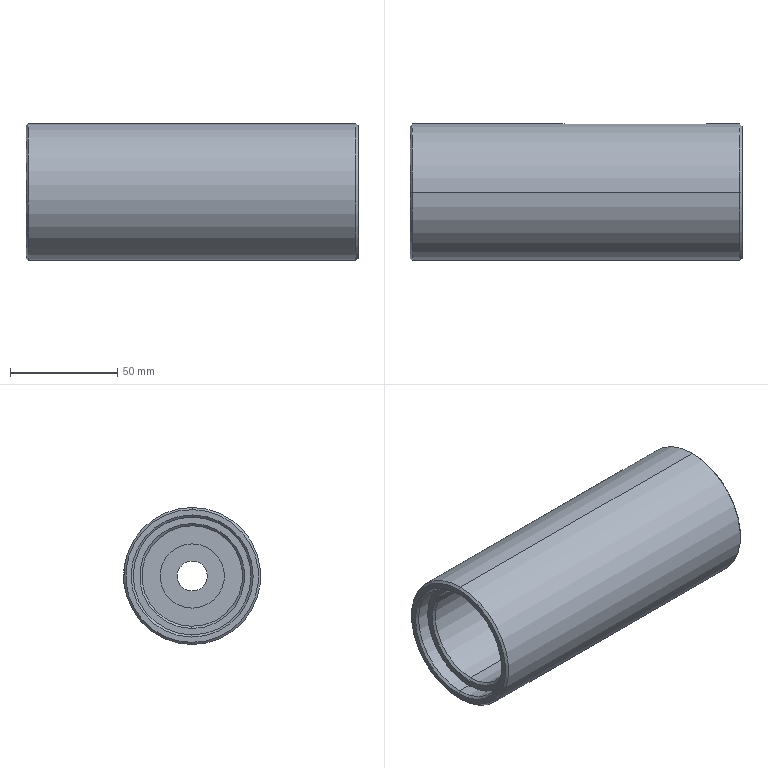Component | SolidWorks | 4-12-12ClampingAxisAssembly-1_4-12-2TelescopicAxis-1 | 1 solid | 28 faces | box 155 x 64 x 64 mm | volume 313641 mm3 | cylinder 12 | cone 8 | plane 8 | commonest cylinder face diameters 14 x2 64 x2 55 x2 47 x2 30 x2 8 x2
build123d program:
from build123d import *

# Parameters (mm, degrees)
HOLE_WIZARD_M16_1_5_D = 14
CHAMFER1_SIZE         = 1
CHAMFER2_SIZE         = 1
CUT_EXTRUDE1_DEPTH    = 4


with BuildPart() as part:
    # Sketch1 → Revolve1 (revolve)
    with BuildSketch(Plane(origin=(0, 0, 0), x_dir=(1, 0, 0), z_dir=(0, 1, 0)), mode=Mode.PRIVATE) as revolve1_sk:
        Polygon((0, 27.5), (0, 32), (155, 32), (155, 0), (104, 0), (104, 15), (94, 15), (94, 23.5), (7, 23.5), (7, 27.5), align=None)
    revolve(revolve1_sk.sketch.rotate(Axis((0, 0, 0), (1, 0, 0)), 180), axis=Axis((0, 0, 0), (1, 0, 0)))

    # Hole Wizard M16 _1.5 (through all)
    with Locations(Plane(origin=(155, 0, 0), x_dir=(0, 0, -1), z_dir=(1, 0, 0))):
        with Locations((0, 0)):
            Hole(HOLE_WIZARD_M16_1_5_D / 2)

    # Chamfer1
    chamfer1_edges = [part.edges().sort_by_distance(p)[0] for p in [
        (0, 0, -32),
        (0, 0, -27.5),
        (7, 0, -23.5),
    ]]
    chamfer(chamfer1_edges, length=CHAMFER1_SIZE)

    # Chamfer2
    chamfer2_edges = [part.edges().sort_by_distance(p)[0] for p in [
        (155, 0, -32),
    ]]
    chamfer(chamfer2_edges, length=CHAMFER2_SIZE)

    # Sketch4 → Cut-Extrude1 (cut)
    with BuildSketch(Plane(origin=(0, 32, 0), x_dir=(-1, 0, 0), z_dir=(0, 1, 0))):
        with BuildLine():
            Line((-136, 4), (-74, 4))
            ThreePointArc((-74, 4), (-70, 0), (-74, -4))
            Line((-74, -4), (-136, -4))
            ThreePointArc((-136, -4), (-140, 0), (-136, 4))
        make_face()
    extrude(amount=-CUT_EXTRUDE1_DEPTH, mode=Mode.SUBTRACT)


solid = part.part

# Placed as in the assembly
solid = solid.moved(Location((-132.809, -4.181, 0), (0.4514, 0, 0)))
STEP:
#1=COLOUR_RGB('',0.7922,0.8196,0.9333);
#2=FILL_AREA_STYLE_COLOUR('',#1);
#3=FILL_AREA_STYLE('',(#2));
#4=SURFACE_STYLE_FILL_AREA(#3);
#5=SURFACE_SIDE_STYLE('',(#4));
#6=SURFACE_STYLE_USAGE(.BOTH.,#5);
#7=PRESENTATION_STYLE_ASSIGNMENT((#6));
#8=CARTESIAN_POINT('',(0.8737,-0.155,-1.22));
#9=VERTEX_POINT('',#8);
#10=CARTESIAN_POINT('',(0.8737,-0.1742,1.22));
#11=VERTEX_POINT('',#10);
#12=CARTESIAN_POINT('',(0.8737,-0.1646,0.));
#13=DIRECTION('',(1.,0.,0.));
#14=DIRECTION('',(0.,-0.007878,1.));
#15=AXIS2_PLACEMENT_3D('',#12,#13,#14);
#16=CIRCLE('',#15,1.22);
#17=EDGE_CURVE('',#9,#11,#16,.T.);
#18=ORIENTED_EDGE('',*,*,#17,.F.);
#19=CARTESIAN_POINT('',(0.8343,-0.1547,-1.26));
#20=VERTEX_POINT('',#19);
#21=CARTESIAN_POINT('',(0.8343,-0.1547,-1.26));
#22=DIRECTION('',(-0.7071,0.005571,-0.7071));
#23=VECTOR('',#22,39.37);
#24=LINE('',#21,#23);
#25=EDGE_CURVE('',#9,#20,#24,.T.);
#26=ORIENTED_EDGE('',*,*,#25,.T.);
#27=CARTESIAN_POINT('',(0.8343,-0.1745,1.26));
#28=VERTEX_POINT('',#27);
#29=CARTESIAN_POINT('',(0.8343,-0.1646,0.));
#30=DIRECTION('',(-1.,-0.,-0.));
#31=DIRECTION('',(0.,-0.007878,1.));
#32=AXIS2_PLACEMENT_3D('',#29,#30,#31);
#33=CIRCLE('',#32,1.26);
#34=EDGE_CURVE('',#28,#20,#33,.T.);
#35=ORIENTED_EDGE('',*,*,#34,.F.);
#36=CARTESIAN_POINT('',(0.8343,-0.1745,1.26));
#37=DIRECTION('',(-0.7071,-0.005571,0.7071));
#38=VECTOR('',#37,39.37);
#39=LINE('',#36,#38);
#40=EDGE_CURVE('',#11,#28,#39,.T.);
#41=ORIENTED_EDGE('',*,*,#40,.F.);
#42=EDGE_LOOP('',(#18,#26,#35,#41));
#43=FACE_OUTER_BOUND('',#42,.T.);
#44=CARTESIAN_POINT('',(0.8343,-0.1646,0.));
#45=DIRECTION('',(-1.,-0.,-0.));
#46=DIRECTION('',(0.,-0.007878,1.));
#47=AXIS2_PLACEMENT_3D('',#44,#45,#46);
#48=CONICAL_SURFACE('',#47,1.26,0.7854);
#49=ADVANCED_FACE('',(#43),#48,.T.);
#50=CARTESIAN_POINT('',(-5.229,-0.1742,1.22));
#51=VERTEX_POINT('',#50);
#52=CARTESIAN_POINT('',(-5.229,-0.155,-1.22));
#53=VERTEX_POINT('',#52);
#54=CARTESIAN_POINT('',(-5.229,-0.1646,0.));
#55=DIRECTION('',(-1.,-0.,-0.));
#56=DIRECTION('',(0.,0.007878,-1.));
#57=AXIS2_PLACEMENT_3D('',#54,#55,#56);
#58=CIRCLE('',#57,1.22);
#59=EDGE_CURVE('',#51,#53,#58,.T.);
#60=ORIENTED_EDGE('',*,*,#59,.F.);
#61=CARTESIAN_POINT('',(-5.189,-0.1745,1.26));
#62=VERTEX_POINT('',#61);
#63=CARTESIAN_POINT('',(-5.229,-0.1742,1.22));
#64=DIRECTION('',(0.7071,-0.005571,0.7071));
#65=VECTOR('',#64,39.37);
#66=LINE('',#63,#65);
#67=EDGE_CURVE('',#51,#62,#66,.T.);
#68=ORIENTED_EDGE('',*,*,#67,.T.);
#69=CARTESIAN_POINT('',(-5.189,-0.1547,-1.26));
#70=VERTEX_POINT('',#69);
#71=CARTESIAN_POINT('',(-5.189,-0.1646,0.));
#72=DIRECTION('',(1.,0.,0.));
#73=DIRECTION('',(0.,0.007878,-1.));
#74=AXIS2_PLACEMENT_3D('',#71,#72,#73);
#75=CIRCLE('',#74,1.26);
#76=EDGE_CURVE('',#70,#62,#75,.T.);
#77=ORIENTED_EDGE('',*,*,#76,.F.);
#78=CARTESIAN_POINT('',(-5.229,-0.155,-1.22));
#79=DIRECTION('',(0.7071,0.005571,-0.7071));
#80=VECTOR('',#79,39.37);
#81=LINE('',#78,#80);
#82=EDGE_CURVE('',#53,#70,#81,.T.);
#83=ORIENTED_EDGE('',*,*,#82,.F.);
#84=EDGE_LOOP('',(#60,#68,#77,#83));
#85=FACE_OUTER_BOUND('',#84,.T.);
#86=CARTESIAN_POINT('',(-5.229,-0.1646,0.));
#87=DIRECTION('',(1.,0.,0.));
#88=DIRECTION('',(0.,0.007878,-1.));
#89=AXIS2_PLACEMENT_3D('',#86,#87,#88);
#90=CONICAL_SURFACE('',#89,1.22,0.7854);
#91=ADVANCED_FACE('',(#85),#90,.T.);
#92=CARTESIAN_POINT('',(-5.189,-0.1561,-1.083));
#93=VERTEX_POINT('',#92);
#94=CARTESIAN_POINT('',(-5.189,-0.1731,1.083));
#95=VERTEX_POINT('',#94);
#96=CARTESIAN_POINT('',(-5.189,-0.1646,0.));
#97=DIRECTION('',(-1.,-0.,-0.));
#98=DIRECTION('',(0.,0.007878,-1.));
#99=AXIS2_PLACEMENT_3D('',#96,#97,#98);
#100=CIRCLE('',#99,1.083);
#101=EDGE_CURVE('',#93,#95,#100,.T.);
#102=ORIENTED_EDGE('',*,*,#101,.F.);
#103=CARTESIAN_POINT('',(-5.229,-0.1558,-1.122));
#104=VERTEX_POINT('',#103);
#105=CARTESIAN_POINT('',(-5.189,-0.1561,-1.083));
#106=DIRECTION('',(-0.7071,0.005571,-0.7071));
#107=VECTOR('',#106,39.37);
#108=LINE('',#105,#107);
#109=EDGE_CURVE('',#93,#104,#108,.T.);
#110=ORIENTED_EDGE('',*,*,#109,.T.);
#111=CARTESIAN_POINT('',(-5.229,-0.1734,1.122));
#112=VERTEX_POINT('',#111);
#113=CARTESIAN_POINT('',(-5.229,-0.1646,0.));
#114=DIRECTION('',(1.,0.,0.));
#115=DIRECTION('',(0.,0.007878,-1.));
#116=AXIS2_PLACEMENT_3D('',#113,#114,#115);
#117=CIRCLE('',#116,1.122);
#118=EDGE_CURVE('',#112,#104,#117,.T.);
#119=ORIENTED_EDGE('',*,*,#118,.F.);
#120=CARTESIAN_POINT('',(-5.189,-0.1731,1.083));
#121=DIRECTION('',(-0.7071,-0.005571,0.7071));
#122=VECTOR('',#121,39.37);
#123=LINE('',#120,#122);
#124=EDGE_CURVE('',#95,#112,#123,.T.);
#125=ORIENTED_EDGE('',*,*,#124,.F.);
#126=EDGE_LOOP('',(#102,#110,#119,#125));
#127=FACE_OUTER_BOUND('',#126,.T.);
#128=CARTESIAN_POINT('',(-5.189,-0.1646,0.));
#129=DIRECTION('',(-1.,-0.,-0.));
#130=DIRECTION('',(0.,-0.007878,1.));
#131=AXIS2_PLACEMENT_3D('',#128,#129,#130);
#132=CONICAL_SURFACE('',#131,1.083,0.7854);
#133=ADVANCED_FACE('',(#127),#132,.F.);
#134=CARTESIAN_POINT('',(-4.914,-0.1573,-0.9252));
#135=VERTEX_POINT('',#134);
#136=CARTESIAN_POINT('',(-4.914,-0.1719,0.9252));
#137=VERTEX_POINT('',#136);
#138=CARTESIAN_POINT('',(-4.914,-0.1646,0.));
#139=DIRECTION('',(-1.,-0.,-0.));
#140=DIRECTION('',(0.,0.007878,-1.));
#141=AXIS2_PLACEMENT_3D('',#138,#139,#140);
#142=CIRCLE('',#141,0.9252);
#143=EDGE_CURVE('',#135,#137,#142,.T.);
#144=ORIENTED_EDGE('',*,*,#143,.F.);
#145=CARTESIAN_POINT('',(-4.953,-0.157,-0.9645));
#146=VERTEX_POINT('',#145);
#147=CARTESIAN_POINT('',(-4.914,-0.1573,-0.9252));
#148=DIRECTION('',(-0.7071,0.005571,-0.7071));
#149=VECTOR('',#148,39.37);
#150=LINE('',#147,#149);
#151=EDGE_CURVE('',#135,#146,#150,.T.);
#152=ORIENTED_EDGE('',*,*,#151,.T.);
#153=CARTESIAN_POINT('',(-4.953,-0.1722,0.9645));
#154=VERTEX_POINT('',#153);
#155=CARTESIAN_POINT('',(-4.953,-0.1646,0.));
#156=DIRECTION('',(1.,0.,0.));
#157=DIRECTION('',(0.,0.007878,-1.));
#158=AXIS2_PLACEMENT_3D('',#155,#156,#157);
#159=CIRCLE('',#158,0.9646);
#160=EDGE_CURVE('',#154,#146,#159,.T.);
#161=ORIENTED_EDGE('',*,*,#160,.F.);
#162=CARTESIAN_POINT('',(-4.914,-0.1719,0.9252));
#163=DIRECTION('',(-0.7071,-0.005571,0.7071));
#164=VECTOR('',#163,39.37);
#165=LINE('',#162,#164);
#166=EDGE_CURVE('',#137,#154,#165,.T.);
#167=ORIENTED_EDGE('',*,*,#166,.F.);
#168=EDGE_LOOP('',(#144,#152,#161,#167));
#169=FACE_OUTER_BOUND('',#168,.T.);
#170=CARTESIAN_POINT('',(-4.914,-0.1646,0.));
#171=DIRECTION('',(-1.,-0.,-0.));
#172=DIRECTION('',(0.,-0.007878,1.));
#173=AXIS2_PLACEMENT_3D('',#170,#171,#172);
#174=CONICAL_SURFACE('',#173,0.9252,0.7854);
#175=ADVANCED_FACE('',(#169),#174,.F.);
#176=CARTESIAN_POINT('',(-1.134,-0.1668,0.2756));
#177=VERTEX_POINT('',#176);
#178=CARTESIAN_POINT('',(-1.134,-0.1624,-0.2756));
#179=VERTEX_POINT('',#178);
#180=CARTESIAN_POINT('',(-1.134,-0.1646,0.));
#181=DIRECTION('',(1.,0.,0.));
#182=DIRECTION('',(0.,0.007878,-1.));
#183=AXIS2_PLACEMENT_3D('',#180,#181,#182);
#184=CIRCLE('',#183,0.2756);
#185=EDGE_CURVE('',#177,#179,#184,.T.);
#186=ORIENTED_EDGE('',*,*,#185,.F.);
#187=CARTESIAN_POINT('',(0.8737,-0.1668,0.2756));
#188=VERTEX_POINT('',#187);
#189=CARTESIAN_POINT('',(0.8737,-0.1668,0.2756));
#190=DIRECTION('',(1.,0.,0.));
#191=VECTOR('',#190,39.37);
#192=LINE('',#189,#191);
#193=EDGE_CURVE('',#177,#188,#192,.T.);
#194=ORIENTED_EDGE('',*,*,#193,.T.);
#195=CARTESIAN_POINT('',(0.8737,-0.1624,-0.2756));
#196=VERTEX_POINT('',#195);
#197=CARTESIAN_POINT('',(0.8737,-0.1646,0.));
#198=DIRECTION('',(1.,0.,0.));
#199=DIRECTION('',(0.,0.007878,-1.));
#200=AXIS2_PLACEMENT_3D('',#197,#198,#199);
#201=CIRCLE('',#200,0.2756);
#202=EDGE_CURVE('',#188,#196,#201,.T.);
#203=ORIENTED_EDGE('',*,*,#202,.T.);
#204=CARTESIAN_POINT('',(0.8737,-0.1624,-0.2756));
#205=DIRECTION('',(1.,0.,0.));
#206=VECTOR('',#205,39.37);
#207=LINE('',#204,#206);
#208=EDGE_CURVE('',#179,#196,#207,.T.);
#209=ORIENTED_EDGE('',*,*,#208,.F.);
#210=EDGE_LOOP('',(#186,#194,#203,#209));
#211=FACE_OUTER_BOUND('',#210,.T.);
#212=CARTESIAN_POINT('',(0.8737,-0.1646,0.));
#213=DIRECTION('',(1.,0.,0.));
#214=DIRECTION('',(0.,0.007878,-1.));
#215=AXIS2_PLACEMENT_3D('',#212,#213,#214);
#216=CYLINDRICAL_SURFACE('',#215,0.2756);
#217=ADVANCED_FACE('',(#211),#216,.F.);
#218=CARTESIAN_POINT('',(0.1256,1.084,0.1673));
#219=VERTEX_POINT('',#218);
#220=CARTESIAN_POINT('',(-2.315,1.084,0.1673));
#221=VERTEX_POINT('',#220);
#222=CARTESIAN_POINT('',(-5.229,1.084,0.1673));
#223=DIRECTION('',(-1.,-0.,-0.));
#224=VECTOR('',#223,39.37);
#225=LINE('',#222,#224);
#226=EDGE_CURVE('',#219,#221,#225,.T.);
#227=ORIENTED_EDGE('',*,*,#226,.T.);
#228=CARTESIAN_POINT('',(-2.315,1.087,-0.1476));
#229=VERTEX_POINT('',#228);
#230=CARTESIAN_POINT('',(-2.315,1.084,0.1673));
#231=CARTESIAN_POINT('',(-2.326,1.084,0.1673));
#232=CARTESIAN_POINT('',(-2.336,1.084,0.1663));
#233=CARTESIAN_POINT('',(-2.356,1.085,0.1623));
#234=CARTESIAN_POINT('',(-2.366,1.085,0.1593));
#235=CARTESIAN_POINT('',(-2.385,1.086,0.1514));
#236=CARTESIAN_POINT('',(-2.394,1.087,0.1465));
#237=CARTESIAN_POINT('',(-2.411,1.088,0.1351));
#238=CARTESIAN_POINT('',(-2.419,1.089,0.1285));
#239=CARTESIAN_POINT('',(-2.434,1.09,0.114));
#240=CARTESIAN_POINT('',(-2.44,1.091,0.1061));
#241=CARTESIAN_POINT('',(-2.452,1.092,0.08887));
#242=CARTESIAN_POINT('',(-2.457,1.093,0.07973));
#243=CARTESIAN_POINT('',(-2.465,1.094,0.0608));
#244=CARTESIAN_POINT('',(-2.468,1.094,0.05087));
#245=CARTESIAN_POINT('',(-2.472,1.095,0.03054));
#246=CARTESIAN_POINT('',(-2.473,1.095,0.02032));
#247=CARTESIAN_POINT('',(-2.473,1.095,-0.0002398));
#248=CARTESIAN_POINT('',(-2.472,1.095,-0.01068));
#249=CARTESIAN_POINT('',(-2.468,1.095,-0.03089));
#250=CARTESIAN_POINT('',(-2.465,1.095,-0.04071));
#251=CARTESIAN_POINT('',(-2.457,1.094,-0.0598));
#252=CARTESIAN_POINT('',(-2.452,1.093,-0.06901));
#253=CARTESIAN_POINT('',(-2.441,1.092,-0.08607));
#254=CARTESIAN_POINT('',(-2.434,1.092,-0.09404));
#255=CARTESIAN_POINT('',(-2.419,1.091,-0.1087));
#256=CARTESIAN_POINT('',(-2.411,1.09,-0.1153));
#257=CARTESIAN_POINT('',(-2.394,1.089,-0.1267));
#258=CARTESIAN_POINT('',(-2.385,1.088,-0.1316));
#259=CARTESIAN_POINT('',(-2.366,1.087,-0.1395));
#260=CARTESIAN_POINT('',(-2.356,1.087,-0.1425));
#261=CARTESIAN_POINT('',(-2.336,1.087,-0.1466));
#262=CARTESIAN_POINT('',(-2.326,1.087,-0.1476));
#263=CARTESIAN_POINT('',(-2.315,1.087,-0.1476));
#264=B_SPLINE_CURVE_WITH_KNOTS('',3,(#230,#231,#232,#233,#234,#235,#236,#237,#238,#239,#240,#241,#242,#243,#244,#245,#246,#247,#248,#249,#250,#251,#252,#253,#254,#255,#256,#257,#258,#259,#260,#261,#262,#263),.UNSPECIFIED.,.F.,.F.,(4,2,2,2,2,2,2,2,2,2,2,2,2,2,2,2,4),(0.,0.0007822,0.001564,0.002347,0.003129,0.003911,0.004693,0.005475,0.006258,0.00704,0.007822,0.008604,0.009386,0.01017,0.01095,0.01173,0.01252),.UNSPECIFIED.);
#265=EDGE_CURVE('',#221,#229,#264,.T.);
#266=ORIENTED_EDGE('',*,*,#265,.T.);
#267=CARTESIAN_POINT('',(0.1256,1.087,-0.1476));
#268=VERTEX_POINT('',#267);
#269=CARTESIAN_POINT('',(-5.229,1.087,-0.1476));
#270=DIRECTION('',(1.,0.,0.));
#271=VECTOR('',#270,39.37);
#272=LINE('',#269,#271);
#273=EDGE_CURVE('',#229,#268,#272,.T.);
#274=ORIENTED_EDGE('',*,*,#273,.T.);
#275=CARTESIAN_POINT('',(0.1256,1.087,-0.1476));
#276=CARTESIAN_POINT('',(0.136,1.087,-0.1476));
#277=CARTESIAN_POINT('',(0.1463,1.087,-0.1466));
#278=CARTESIAN_POINT('',(0.1664,1.087,-0.1426));
#279=CARTESIAN_POINT('',(0.1764,1.087,-0.1396));
#280=CARTESIAN_POINT('',(0.1955,1.088,-0.1316));
#281=CARTESIAN_POINT('',(0.2045,1.089,-0.1268));
#282=CARTESIAN_POINT('',(0.2216,1.09,-0.1154));
#283=CARTESIAN_POINT('',(0.2297,1.091,-0.1087));
#284=CARTESIAN_POINT('',(0.2442,1.092,-0.0942));
#285=CARTESIAN_POINT('',(0.2508,1.092,-0.08628));
#286=CARTESIAN_POINT('',(0.2623,1.093,-0.06906));
#287=CARTESIAN_POINT('',(0.2672,1.094,-0.05991));
#288=CARTESIAN_POINT('',(0.275,1.095,-0.04096));
#289=CARTESIAN_POINT('',(0.278,1.095,-0.03103));
#290=CARTESIAN_POINT('',(0.2821,1.095,-0.01069));
#291=CARTESIAN_POINT('',(0.2831,1.095,-0.0004692));
#292=CARTESIAN_POINT('',(0.2831,1.095,0.02009));
#293=CARTESIAN_POINT('',(0.2821,1.095,0.03053));
#294=CARTESIAN_POINT('',(0.2781,1.094,0.05073));
#295=CARTESIAN_POINT('',(0.2751,1.094,0.06055));
#296=CARTESIAN_POINT('',(0.2672,1.093,0.07962));
#297=CARTESIAN_POINT('',(0.2623,1.092,0.08882));
#298=CARTESIAN_POINT('',(0.2509,1.091,0.1059));
#299=CARTESIAN_POINT('',(0.2444,1.09,0.1138));
#300=CARTESIAN_POINT('',(0.2297,1.089,0.1285));
#301=CARTESIAN_POINT('',(0.2218,1.088,0.135));
#302=CARTESIAN_POINT('',(0.2047,1.087,0.1464));
#303=CARTESIAN_POINT('',(0.1955,1.086,0.1514));
#304=CARTESIAN_POINT('',(0.1765,1.085,0.1593));
#305=CARTESIAN_POINT('',(0.1667,1.085,0.1622));
#306=CARTESIAN_POINT('',(0.1465,1.084,0.1663));
#307=CARTESIAN_POINT('',(0.136,1.084,0.1673));
#308=CARTESIAN_POINT('',(0.1256,1.084,0.1673));
#309=B_SPLINE_CURVE_WITH_KNOTS('',3,(#275,#276,#277,#278,#279,#280,#281,#282,#283,#284,#285,#286,#287,#288,#289,#290,#291,#292,#293,#294,#295,#296,#297,#298,#299,#300,#301,#302,#303,#304,#305,#306,#307,#308),.UNSPECIFIED.,.F.,.F.,(4,2,2,2,2,2,2,2,2,2,2,2,2,2,2,2,4),(0.,0.0007822,0.001564,0.002347,0.003129,0.003911,0.004693,0.005475,0.006258,0.00704,0.007822,0.008604,0.009386,0.01017,0.01095,0.01173,0.01252),.UNSPECIFIED.);
#310=EDGE_CURVE('',#268,#219,#309,.T.);
#311=ORIENTED_EDGE('',*,*,#310,.T.);
#312=EDGE_LOOP('',(#227,#266,#274,#311));
#313=FACE_BOUND('',#312,.T.);
#314=ORIENTED_EDGE('',*,*,#34,.T.);
#315=CARTESIAN_POINT('',(-5.229,-0.1547,-1.26));
#316=DIRECTION('',(-1.,-0.,-0.));
#317=VECTOR('',#316,39.37);
#318=LINE('',#315,#317);
#319=EDGE_CURVE('',#20,#70,#318,.T.);
#320=ORIENTED_EDGE('',*,*,#319,.T.);
#321=ORIENTED_EDGE('',*,*,#76,.T.);
#322=CARTESIAN_POINT('',(-5.229,-0.1745,1.26));
#323=DIRECTION('',(-1.,-0.,-0.));
#324=VECTOR('',#323,39.37);
#325=LINE('',#322,#324);
#326=EDGE_CURVE('',#28,#62,#325,.T.);
#327=ORIENTED_EDGE('',*,*,#326,.F.);
#328=EDGE_LOOP('',(#314,#320,#321,#327));
#329=FACE_OUTER_BOUND('',#328,.T.);
#330=CARTESIAN_POINT('',(-5.229,-0.1646,0.));
#331=DIRECTION('',(-1.,-0.,-0.));
#332=DIRECTION('',(0.,-0.007878,1.));
#333=AXIS2_PLACEMENT_3D('',#330,#331,#332);
#334=CYLINDRICAL_SURFACE('',#333,1.26);
#335=ADVANCED_FACE('',(#313,#329),#334,.T.);
#336=CARTESIAN_POINT('',(-4.953,-0.1561,-1.083));
#337=VERTEX_POINT('',#336);
#338=CARTESIAN_POINT('',(-4.953,-0.1731,1.083));
#339=VERTEX_POINT('',#338);
#340=CARTESIAN_POINT('',(-4.953,-0.1646,0.));
#341=DIRECTION('',(-1.,-0.,-0.));
#342=DIRECTION('',(0.,-0.007878,1.));
#343=AXIS2_PLACEMENT_3D('',#340,#341,#342);
#344=CIRCLE('',#343,1.083);
#345=EDGE_CURVE('',#337,#339,#344,.T.);
#346=ORIENTED_EDGE('',*,*,#345,.F.);
#347=CARTESIAN_POINT('',(-5.229,-0.1561,-1.083));
#348=DIRECTION('',(-1.,-0.,-0.));
#349=VECTOR('',#348,39.37);
#350=LINE('',#347,#349);
#351=EDGE_CURVE('',#337,#93,#350,.T.);
#352=ORIENTED_EDGE('',*,*,#351,.T.);
#353=ORIENTED_EDGE('',*,*,#101,.T.);
#354=CARTESIAN_POINT('',(-5.229,-0.1731,1.083));
#355=DIRECTION('',(-1.,-0.,-0.));
#356=VECTOR('',#355,39.37);
#357=LINE('',#354,#356);
#358=EDGE_CURVE('',#339,#95,#357,.T.);
#359=ORIENTED_EDGE('',*,*,#358,.F.);
#360=EDGE_LOOP('',(#346,#352,#353,#359));
#361=FACE_OUTER_BOUND('',#360,.T.);
#362=CARTESIAN_POINT('',(-5.229,-0.1646,0.));
#363=DIRECTION('',(-1.,-0.,-0.));
#364=DIRECTION('',(0.,-0.007878,1.));
#365=AXIS2_PLACEMENT_3D('',#362,#363,#364);
#366=CYLINDRICAL_SURFACE('',#365,1.083);
#367=ADVANCED_FACE('',(#361),#366,.F.);
#368=CARTESIAN_POINT('',(-1.528,-0.1573,-0.9252));
#369=VERTEX_POINT('',#368);
#370=CARTESIAN_POINT('',(-1.528,-0.1719,0.9252));
#371=VERTEX_POINT('',#370);
#372=CARTESIAN_POINT('',(-1.528,-0.1646,0.));
#373=DIRECTION('',(-1.,-0.,-0.));
#374=DIRECTION('',(0.,-0.007878,1.));
#375=AXIS2_PLACEMENT_3D('',#372,#373,#374);
#376=CIRCLE('',#375,0.9252);
#377=EDGE_CURVE('',#369,#371,#376,.T.);
#378=ORIENTED_EDGE('',*,*,#377,.F.);
#379=CARTESIAN_POINT('',(-5.229,-0.1573,-0.9252));
#380=DIRECTION('',(-1.,-0.,-0.));
#381=VECTOR('',#380,39.37);
#382=LINE('',#379,#381);
#383=EDGE_CURVE('',#369,#135,#382,.T.);
#384=ORIENTED_EDGE('',*,*,#383,.T.);
#385=ORIENTED_EDGE('',*,*,#143,.T.);
#386=CARTESIAN_POINT('',(-5.229,-0.1719,0.9252));
#387=DIRECTION('',(-1.,-0.,-0.));
#388=VECTOR('',#387,39.37);
#389=LINE('',#386,#388);
#390=EDGE_CURVE('',#371,#137,#389,.T.);
#391=ORIENTED_EDGE('',*,*,#390,.F.);
#392=EDGE_LOOP('',(#378,#384,#385,#391));
#393=FACE_OUTER_BOUND('',#392,.T.);
#394=CARTESIAN_POINT('',(-5.229,-0.1646,0.));
#395=DIRECTION('',(-1.,-0.,-0.));
#396=DIRECTION('',(0.,-0.007878,1.));
#397=AXIS2_PLACEMENT_3D('',#394,#395,#396);
#398=CYLINDRICAL_SURFACE('',#397,0.9252);
#399=ADVANCED_FACE('',(#393),#398,.F.);
#400=CARTESIAN_POINT('',(-1.134,-0.16,-0.5905));
#401=VERTEX_POINT('',#400);
#402=CARTESIAN_POINT('',(-1.134,-0.1693,0.5905));
#403=VERTEX_POINT('',#402);
#404=CARTESIAN_POINT('',(-1.134,-0.1646,0.));
#405=DIRECTION('',(-1.,-0.,-0.));
#406=DIRECTION('',(0.,-0.007878,1.));
#407=AXIS2_PLACEMENT_3D('',#404,#405,#406);
#408=CIRCLE('',#407,0.5906);
#409=EDGE_CURVE('',#401,#403,#408,.T.);
#410=ORIENTED_EDGE('',*,*,#409,.F.);
#411=CARTESIAN_POINT('',(-1.528,-0.16,-0.5905));
#412=VERTEX_POINT('',#411);
#413=CARTESIAN_POINT('',(-5.229,-0.16,-0.5905));
#414=DIRECTION('',(-1.,-0.,-0.));
#415=VECTOR('',#414,39.37);
#416=LINE('',#413,#415);
#417=EDGE_CURVE('',#401,#412,#416,.T.);
#418=ORIENTED_EDGE('',*,*,#417,.T.);
#419=CARTESIAN_POINT('',(-1.528,-0.1693,0.5905));
#420=VERTEX_POINT('',#419);
#421=CARTESIAN_POINT('',(-1.528,-0.1646,0.));
#422=DIRECTION('',(-1.,-0.,-0.));
#423=DIRECTION('',(0.,-0.007878,1.));
#424=AXIS2_PLACEMENT_3D('',#421,#422,#423);
#425=CIRCLE('',#424,0.5906);
#426=EDGE_CURVE('',#412,#420,#425,.T.);
#427=ORIENTED_EDGE('',*,*,#426,.T.);
#428=CARTESIAN_POINT('',(-5.229,-0.1693,0.5905));
#429=DIRECTION('',(-1.,-0.,-0.));
#430=VECTOR('',#429,39.37);
#431=LINE('',#428,#430);
#432=EDGE_CURVE('',#403,#420,#431,.T.);
#433=ORIENTED_EDGE('',*,*,#432,.F.);
#434=EDGE_LOOP('',(#410,#418,#427,#433));
#435=FACE_OUTER_BOUND('',#434,.T.);
#436=CARTESIAN_POINT('',(-5.229,-0.1646,0.));
#437=DIRECTION('',(-1.,-0.,-0.));
#438=DIRECTION('',(0.,-0.007878,1.));
#439=AXIS2_PLACEMENT_3D('',#436,#437,#438);
#440=CYLINDRICAL_SURFACE('',#439,0.5906);
#441=ADVANCED_FACE('',(#435),#440,.F.);
#442=CARTESIAN_POINT('',(-1.134,-0.1646,0.));
#443=DIRECTION('',(1.,0.,0.));
#444=DIRECTION('',(0.,0.007878,-1.));
#445=AXIS2_PLACEMENT_3D('',#442,#443,#444);
#446=CIRCLE('',#445,0.2756);
#447=EDGE_CURVE('',#179,#177,#446,.T.);
#448=ORIENTED_EDGE('',*,*,#447,.T.);
#449=ORIENTED_EDGE('',*,*,#185,.T.);
#450=EDGE_LOOP('',(#448,#449));
#451=FACE_BOUND('',#450,.T.);
#452=CARTESIAN_POINT('',(-1.134,-0.1646,0.));
#453=DIRECTION('',(-1.,-0.,-0.));
#454=DIRECTION('',(0.,-0.007878,1.));
#455=AXIS2_PLACEMENT_3D('',#452,#453,#454);
#456=CIRCLE('',#455,0.5906);
#457=EDGE_CURVE('',#403,#401,#456,.T.);
#458=ORIENTED_EDGE('',*,*,#457,.T.);
#459=ORIENTED_EDGE('',*,*,#409,.T.);
#460=EDGE_LOOP('',(#458,#459));
#461=FACE_OUTER_BOUND('',#460,.T.);
#462=CARTESIAN_POINT('',(-1.134,-0.1646,0.));
#463=DIRECTION('',(1.,0.,0.));
#464=DIRECTION('',(0.,0.007878,-1.));
#465=AXIS2_PLACEMENT_3D('',#462,#463,#464);
#466=PLANE('',#465);
#467=ADVANCED_FACE('',(#451,#461),#466,.F.);
#468=ORIENTED_EDGE('',*,*,#417,.F.);
#469=ORIENTED_EDGE('',*,*,#457,.F.);
#470=ORIENTED_EDGE('',*,*,#432,.T.);
#471=CARTESIAN_POINT('',(-1.528,-0.1646,0.));
#472=DIRECTION('',(-1.,-0.,-0.));
#473=DIRECTION('',(0.,-0.007878,1.));
#474=AXIS2_PLACEMENT_3D('',#471,#472,#473);
#475=CIRCLE('',#474,0.5906);
#476=EDGE_CURVE('',#420,#412,#475,.T.);
#477=ORIENTED_EDGE('',*,*,#476,.T.);
#478=EDGE_LOOP('',(#468,#469,#470,#477));
#479=FACE_OUTER_BOUND('',#478,.T.);
#480=CARTESIAN_POINT('',(-5.229,-0.1646,0.));
#481=DIRECTION('',(-1.,-0.,-0.));
#482=DIRECTION('',(0.,-0.007878,1.));
#483=AXIS2_PLACEMENT_3D('',#480,#481,#482);
#484=CYLINDRICAL_SURFACE('',#483,0.5906);
#485=ADVANCED_FACE('',(#479),#484,.F.);
#486=ORIENTED_EDGE('',*,*,#476,.F.);
#487=ORIENTED_EDGE('',*,*,#426,.F.);
#488=EDGE_LOOP('',(#486,#487));
#489=FACE_BOUND('',#488,.T.);
#490=CARTESIAN_POINT('',(-1.528,-0.1646,0.));
#491=DIRECTION('',(-1.,-0.,-0.));
#492=DIRECTION('',(0.,-0.007878,1.));
#493=AXIS2_PLACEMENT_3D('',#490,#491,#492);
#494=CIRCLE('',#493,0.9252);
#495=EDGE_CURVE('',#371,#369,#494,.T.);
#496=ORIENTED_EDGE('',*,*,#495,.T.);
#497=ORIENTED_EDGE('',*,*,#377,.T.);
#498=EDGE_LOOP('',(#496,#497));
#499=FACE_OUTER_BOUND('',#498,.T.);
#500=CARTESIAN_POINT('',(-1.528,-0.16,-0.5905));
#501=DIRECTION('',(1.,0.,0.));
#502=DIRECTION('',(0.,0.007878,-1.));
#503=AXIS2_PLACEMENT_3D('',#500,#501,#502);
#504=PLANE('',#503);
#505=ADVANCED_FACE('',(#489,#499),#504,.F.);
#506=ORIENTED_EDGE('',*,*,#383,.F.);
#507=ORIENTED_EDGE('',*,*,#495,.F.);
#508=ORIENTED_EDGE('',*,*,#390,.T.);
#509=CARTESIAN_POINT('',(-4.914,-0.1646,0.));
#510=DIRECTION('',(-1.,-0.,-0.));
#511=DIRECTION('',(0.,0.007878,-1.));
#512=AXIS2_PLACEMENT_3D('',#509,#510,#511);
#513=CIRCLE('',#512,0.9252);
#514=EDGE_CURVE('',#137,#135,#513,.T.);
#515=ORIENTED_EDGE('',*,*,#514,.T.);
#516=EDGE_LOOP('',(#506,#507,#508,#515));
#517=FACE_OUTER_BOUND('',#516,.T.);
#518=CARTESIAN_POINT('',(-5.229,-0.1646,0.));
#519=DIRECTION('',(-1.,-0.,-0.));
#520=DIRECTION('',(0.,-0.007878,1.));
#521=AXIS2_PLACEMENT_3D('',#518,#519,#520);
#522=CYLINDRICAL_SURFACE('',#521,0.9252);
#523=ADVANCED_FACE('',(#517),#522,.F.);
#524=ORIENTED_EDGE('',*,*,#160,.T.);
#525=CARTESIAN_POINT('',(-4.953,-0.1646,0.));
#526=DIRECTION('',(1.,0.,0.));
#527=DIRECTION('',(0.,0.007878,-1.));
#528=AXIS2_PLACEMENT_3D('',#525,#526,#527);
#529=CIRCLE('',#528,0.9646);
#530=EDGE_CURVE('',#146,#154,#529,.T.);
#531=ORIENTED_EDGE('',*,*,#530,.T.);
#532=EDGE_LOOP('',(#524,#531));
#533=FACE_BOUND('',#532,.T.);
#534=CARTESIAN_POINT('',(-4.953,-0.1646,0.));
#535=DIRECTION('',(-1.,-0.,-0.));
#536=DIRECTION('',(0.,-0.007878,1.));
#537=AXIS2_PLACEMENT_3D('',#534,#535,#536);
#538=CIRCLE('',#537,1.083);
#539=EDGE_CURVE('',#339,#337,#538,.T.);
#540=ORIENTED_EDGE('',*,*,#539,.T.);
#541=ORIENTED_EDGE('',*,*,#345,.T.);
#542=EDGE_LOOP('',(#540,#541));
#543=FACE_OUTER_BOUND('',#542,.T.);
#544=CARTESIAN_POINT('',(-4.953,-0.1573,-0.9252));
#545=DIRECTION('',(1.,0.,0.));
#546=DIRECTION('',(0.,0.007878,-1.));
#547=AXIS2_PLACEMENT_3D('',#544,#545,#546);
#548=PLANE('',#547);
#549=ADVANCED_FACE('',(#533,#543),#548,.F.);
#550=ORIENTED_EDGE('',*,*,#351,.F.);
#551=ORIENTED_EDGE('',*,*,#539,.F.);
#552=ORIENTED_EDGE('',*,*,#358,.T.);
#553=CARTESIAN_POINT('',(-5.189,-0.1646,0.));
#554=DIRECTION('',(-1.,-0.,-0.));
#555=DIRECTION('',(0.,0.007878,-1.));
#556=AXIS2_PLACEMENT_3D('',#553,#554,#555);
#557=CIRCLE('',#556,1.083);
#558=EDGE_CURVE('',#95,#93,#557,.T.);
#559=ORIENTED_EDGE('',*,*,#558,.T.);
#560=EDGE_LOOP('',(#550,#551,#552,#559));
#561=FACE_OUTER_BOUND('',#560,.T.);
#562=CARTESIAN_POINT('',(-5.229,-0.1646,0.));
#563=DIRECTION('',(-1.,-0.,-0.));
#564=DIRECTION('',(0.,-0.007878,1.));
#565=AXIS2_PLACEMENT_3D('',#562,#563,#564);
#566=CYLINDRICAL_SURFACE('',#565,1.083);
#567=ADVANCED_FACE('',(#561),#566,.F.);
#568=ORIENTED_EDGE('',*,*,#118,.T.);
#569=CARTESIAN_POINT('',(-5.229,-0.1646,0.));
#570=DIRECTION('',(1.,0.,0.));
#571=DIRECTION('',(0.,0.007878,-1.));
#572=AXIS2_PLACEMENT_3D('',#569,#570,#571);
#573=CIRCLE('',#572,1.122);
#574=EDGE_CURVE('',#104,#112,#573,.T.);
#575=ORIENTED_EDGE('',*,*,#574,.T.);
#576=EDGE_LOOP('',(#568,#575));
#577=FACE_BOUND('',#576,.T.);
#578=CARTESIAN_POINT('',(-5.229,-0.1646,0.));
#579=DIRECTION('',(-1.,-0.,-0.));
#580=DIRECTION('',(0.,0.007878,-1.));
#581=AXIS2_PLACEMENT_3D('',#578,#579,#580);
#582=CIRCLE('',#581,1.22);
#583=EDGE_CURVE('',#53,#51,#582,.T.);
#584=ORIENTED_EDGE('',*,*,#583,.T.);
#585=ORIENTED_EDGE('',*,*,#59,.T.);
#586=EDGE_LOOP('',(#584,#585));
#587=FACE_OUTER_BOUND('',#586,.T.);
#588=CARTESIAN_POINT('',(-5.229,-0.1561,-1.083));
#589=DIRECTION('',(1.,0.,0.));
#590=DIRECTION('',(0.,0.007878,-1.));
#591=AXIS2_PLACEMENT_3D('',#588,#589,#590);
#592=PLANE('',#591);
#593=ADVANCED_FACE('',(#577,#587),#592,.F.);
#594=ORIENTED_EDGE('',*,*,#319,.F.);
#595=CARTESIAN_POINT('',(0.8343,-0.1646,0.));
#596=DIRECTION('',(-1.,-0.,-0.));
#597=DIRECTION('',(0.,-0.007878,1.));
#598=AXIS2_PLACEMENT_3D('',#595,#596,#597);
#599=CIRCLE('',#598,1.26);
#600=EDGE_CURVE('',#20,#28,#599,.T.);
#601=ORIENTED_EDGE('',*,*,#600,.T.);
#602=ORIENTED_EDGE('',*,*,#326,.T.);
#603=CARTESIAN_POINT('',(-5.189,-0.1646,0.));
#604=DIRECTION('',(1.,0.,0.));
#605=DIRECTION('',(0.,0.007878,-1.));
#606=AXIS2_PLACEMENT_3D('',#603,#604,#605);
#607=CIRCLE('',#606,1.26);
#608=EDGE_CURVE('',#62,#70,#607,.T.);
#609=ORIENTED_EDGE('',*,*,#608,.T.);
#610=EDGE_LOOP('',(#594,#601,#602,#609));
#611=FACE_OUTER_BOUND('',#610,.T.);
#612=CARTESIAN_POINT('',(-5.229,-0.1646,0.));
#613=DIRECTION('',(-1.,-0.,-0.));
#614=DIRECTION('',(0.,-0.007878,1.));
#615=AXIS2_PLACEMENT_3D('',#612,#613,#614);
#616=CYLINDRICAL_SURFACE('',#615,1.26);
#617=ADVANCED_FACE('',(#611),#616,.T.);
#618=CARTESIAN_POINT('',(0.8737,-0.1646,0.));
#619=DIRECTION('',(1.,0.,0.));
#620=DIRECTION('',(0.,-0.007878,1.));
#621=AXIS2_PLACEMENT_3D('',#618,#619,#620);
#622=CIRCLE('',#621,1.22);
#623=EDGE_CURVE('',#11,#9,#622,.T.);
#624=ORIENTED_EDGE('',*,*,#623,.T.);
#625=ORIENTED_EDGE('',*,*,#17,.T.);
#626=EDGE_LOOP('',(#624,#625));
#627=FACE_OUTER_BOUND('',#626,.T.);
#628=CARTESIAN_POINT('',(0.8737,-0.1646,0.));
#629=DIRECTION('',(1.,0.,0.));
#630=DIRECTION('',(0.,0.007878,-1.));
#631=AXIS2_PLACEMENT_3D('',#628,#629,#630);
#632=CIRCLE('',#631,0.2756);
#633=EDGE_CURVE('',#196,#188,#632,.T.);
#634=ORIENTED_EDGE('',*,*,#633,.F.);
#635=ORIENTED_EDGE('',*,*,#202,.F.);
#636=EDGE_LOOP('',(#634,#635));
#637=FACE_BOUND('',#636,.T.);
#638=CARTESIAN_POINT('',(0.8737,-0.1547,-1.26));
#639=DIRECTION('',(-1.,-0.,-0.));
#640=DIRECTION('',(-0.,-0.007878,1.));
#641=AXIS2_PLACEMENT_3D('',#638,#639,#640);
#642=PLANE('',#641);
#643=ADVANCED_FACE('',(#627,#637),#642,.F.);
#644=ORIENTED_EDGE('',*,*,#193,.F.);
#645=ORIENTED_EDGE('',*,*,#447,.F.);
#646=ORIENTED_EDGE('',*,*,#208,.T.);
#647=ORIENTED_EDGE('',*,*,#633,.T.);
#648=EDGE_LOOP('',(#644,#645,#646,#647));
#649=FACE_OUTER_BOUND('',#648,.T.);
#650=CARTESIAN_POINT('',(0.8737,-0.1646,0.));
#651=DIRECTION('',(1.,0.,0.));
#652=DIRECTION('',(0.,0.007878,-1.));
#653=AXIS2_PLACEMENT_3D('',#650,#651,#652);
#654=CYLINDRICAL_SURFACE('',#653,0.2756);
#655=ADVANCED_FACE('',(#649),#654,.F.);
#656=ORIENTED_EDGE('',*,*,#151,.F.);
#657=ORIENTED_EDGE('',*,*,#514,.F.);
#658=ORIENTED_EDGE('',*,*,#166,.T.);
#659=ORIENTED_EDGE('',*,*,#530,.F.);
#660=EDGE_LOOP('',(#656,#657,#658,#659));
#661=FACE_OUTER_BOUND('',#660,.T.);
#662=CARTESIAN_POINT('',(-4.914,-0.1646,0.));
#663=DIRECTION('',(-1.,-0.,-0.));
#664=DIRECTION('',(0.,-0.007878,1.));
#665=AXIS2_PLACEMENT_3D('',#662,#663,#664);
#666=CONICAL_SURFACE('',#665,0.9252,0.7854);
#667=ADVANCED_FACE('',(#661),#666,.F.);
#668=ORIENTED_EDGE('',*,*,#109,.F.);
#669=ORIENTED_EDGE('',*,*,#558,.F.);
#670=ORIENTED_EDGE('',*,*,#124,.T.);
#671=ORIENTED_EDGE('',*,*,#574,.F.);
#672=EDGE_LOOP('',(#668,#669,#670,#671));
#673=FACE_OUTER_BOUND('',#672,.T.);
#674=CARTESIAN_POINT('',(-5.189,-0.1646,0.));
#675=DIRECTION('',(-1.,-0.,-0.));
#676=DIRECTION('',(0.,-0.007878,1.));
#677=AXIS2_PLACEMENT_3D('',#674,#675,#676);
#678=CONICAL_SURFACE('',#677,1.083,0.7854);
#679=ADVANCED_FACE('',(#673),#678,.F.);
#680=ORIENTED_EDGE('',*,*,#67,.F.);
#681=ORIENTED_EDGE('',*,*,#583,.F.);
#682=ORIENTED_EDGE('',*,*,#82,.T.);
#683=ORIENTED_EDGE('',*,*,#608,.F.);
#684=EDGE_LOOP('',(#680,#681,#682,#683));
#685=FACE_OUTER_BOUND('',#684,.T.);
#686=CARTESIAN_POINT('',(-5.229,-0.1646,0.));
#687=DIRECTION('',(1.,0.,0.));
#688=DIRECTION('',(0.,0.007878,-1.));
#689=AXIS2_PLACEMENT_3D('',#686,#687,#688);
#690=CONICAL_SURFACE('',#689,1.22,0.7854);
#691=ADVANCED_FACE('',(#685),#690,.T.);
#692=ORIENTED_EDGE('',*,*,#25,.F.);
#693=ORIENTED_EDGE('',*,*,#623,.F.);
#694=ORIENTED_EDGE('',*,*,#40,.T.);
#695=ORIENTED_EDGE('',*,*,#600,.F.);
#696=EDGE_LOOP('',(#692,#693,#694,#695));
#697=FACE_OUTER_BOUND('',#696,.T.);
#698=CARTESIAN_POINT('',(0.8343,-0.1646,0.));
#699=DIRECTION('',(-1.,-0.,-0.));
#700=DIRECTION('',(0.,-0.007878,1.));
#701=AXIS2_PLACEMENT_3D('',#698,#699,#700);
#702=CONICAL_SURFACE('',#701,1.26,0.7854);
#703=ADVANCED_FACE('',(#697),#702,.T.);
#704=CARTESIAN_POINT('',(0.1256,0.939,-0.1488));
#705=VERTEX_POINT('',#704);
#706=CARTESIAN_POINT('',(0.1256,0.939,-0.1488));
#707=DIRECTION('',(-0.,1.,0.007878));
#708=VECTOR('',#707,39.37);
#709=LINE('',#706,#708);
#710=EDGE_CURVE('',#705,#268,#709,.T.);
#711=ORIENTED_EDGE('',*,*,#710,.F.);
#712=CARTESIAN_POINT('',(0.1256,0.9365,0.1662));
#713=VERTEX_POINT('',#712);
#714=CARTESIAN_POINT('',(0.1256,0.9377,0.008685));
#715=DIRECTION('',(-0.,1.,0.007878));
#716=DIRECTION('',(0.,-0.007878,1.));
#717=AXIS2_PLACEMENT_3D('',#714,#715,#716);
#718=CIRCLE('',#717,0.1575);
#719=EDGE_CURVE('',#713,#705,#718,.T.);
#720=ORIENTED_EDGE('',*,*,#719,.F.);
#721=CARTESIAN_POINT('',(0.1256,0.9365,0.1662));
#722=DIRECTION('',(-0.,1.,0.007878));
#723=VECTOR('',#722,39.37);
#724=LINE('',#721,#723);
#725=EDGE_CURVE('',#713,#219,#724,.T.);
#726=ORIENTED_EDGE('',*,*,#725,.T.);
#727=ORIENTED_EDGE('',*,*,#310,.F.);
#728=EDGE_LOOP('',(#711,#720,#726,#727));
#729=FACE_OUTER_BOUND('',#728,.T.);
#730=CARTESIAN_POINT('',(0.1256,0.9377,0.008685));
#731=DIRECTION('',(-0.,1.,0.007878));
#732=DIRECTION('',(0.,-0.007878,1.));
#733=AXIS2_PLACEMENT_3D('',#730,#731,#732);
#734=CYLINDRICAL_SURFACE('',#733,0.1575);
#735=ADVANCED_FACE('',(#729),#734,.F.);
#736=ORIENTED_EDGE('',*,*,#725,.F.);
#737=CARTESIAN_POINT('',(-2.315,0.9365,0.1662));
#738=VERTEX_POINT('',#737);
#739=CARTESIAN_POINT('',(0.1256,0.9365,0.1662));
#740=DIRECTION('',(1.,0.,-0.));
#741=VECTOR('',#740,39.37);
#742=LINE('',#739,#741);
#743=EDGE_CURVE('',#738,#713,#742,.T.);
#744=ORIENTED_EDGE('',*,*,#743,.F.);
#745=CARTESIAN_POINT('',(-2.315,0.9365,0.1662));
#746=DIRECTION('',(-0.,1.,0.007878));
#747=VECTOR('',#746,39.37);
#748=LINE('',#745,#747);
#749=EDGE_CURVE('',#738,#221,#748,.T.);
#750=ORIENTED_EDGE('',*,*,#749,.T.);
#751=ORIENTED_EDGE('',*,*,#226,.F.);
#752=EDGE_LOOP('',(#736,#744,#750,#751));
#753=FACE_OUTER_BOUND('',#752,.T.);
#754=CARTESIAN_POINT('',(0.1256,0.9365,0.1662));
#755=DIRECTION('',(0.,-0.007878,1.));
#756=DIRECTION('',(1.,0.,-0.));
#757=AXIS2_PLACEMENT_3D('',#754,#755,#756);
#758=PLANE('',#757);
#759=ADVANCED_FACE('',(#753),#758,.F.);
#760=ORIENTED_EDGE('',*,*,#749,.F.);
#761=CARTESIAN_POINT('',(-2.315,0.939,-0.1488));
#762=VERTEX_POINT('',#761);
#763=CARTESIAN_POINT('',(-2.315,0.9377,0.008685));
#764=DIRECTION('',(-0.,1.,0.007878));
#765=DIRECTION('',(0.,-0.007878,1.));
#766=AXIS2_PLACEMENT_3D('',#763,#764,#765);
#767=CIRCLE('',#766,0.1575);
#768=EDGE_CURVE('',#762,#738,#767,.T.);
#769=ORIENTED_EDGE('',*,*,#768,.F.);
#770=CARTESIAN_POINT('',(-2.315,0.939,-0.1488));
#771=DIRECTION('',(-0.,1.,0.007878));
#772=VECTOR('',#771,39.37);
#773=LINE('',#770,#772);
#774=EDGE_CURVE('',#762,#229,#773,.T.);
#775=ORIENTED_EDGE('',*,*,#774,.T.);
#776=ORIENTED_EDGE('',*,*,#265,.F.);
#777=EDGE_LOOP('',(#760,#769,#775,#776));
#778=FACE_OUTER_BOUND('',#777,.T.);
#779=CARTESIAN_POINT('',(-2.315,0.9377,0.008685));
#780=DIRECTION('',(-0.,1.,0.007878));
#781=DIRECTION('',(0.,-0.007878,1.));
#782=AXIS2_PLACEMENT_3D('',#779,#780,#781);
#783=CYLINDRICAL_SURFACE('',#782,0.1575);
#784=ADVANCED_FACE('',(#778),#783,.F.);
#785=ORIENTED_EDGE('',*,*,#774,.F.);
#786=CARTESIAN_POINT('',(-2.315,0.939,-0.1488));
#787=DIRECTION('',(-1.,-0.,0.));
#788=VECTOR('',#787,39.37);
#789=LINE('',#786,#788);
#790=EDGE_CURVE('',#705,#762,#789,.T.);
#791=ORIENTED_EDGE('',*,*,#790,.F.);
#792=ORIENTED_EDGE('',*,*,#710,.T.);
#793=ORIENTED_EDGE('',*,*,#273,.F.);
#794=EDGE_LOOP('',(#785,#791,#792,#793));
#795=FACE_OUTER_BOUND('',#794,.T.);
#796=CARTESIAN_POINT('',(-2.315,0.939,-0.1488));
#797=DIRECTION('',(-0.,0.007878,-1.));
#798=DIRECTION('',(-1.,-0.,0.));
#799=AXIS2_PLACEMENT_3D('',#796,#797,#798);
#800=PLANE('',#799);
#801=ADVANCED_FACE('',(#795),#800,.F.);
#802=ORIENTED_EDGE('',*,*,#719,.T.);
#803=ORIENTED_EDGE('',*,*,#790,.T.);
#804=ORIENTED_EDGE('',*,*,#768,.T.);
#805=ORIENTED_EDGE('',*,*,#743,.T.);
#806=EDGE_LOOP('',(#802,#803,#804,#805));
#807=FACE_OUTER_BOUND('',#806,.T.);
#808=CARTESIAN_POINT('',(0.1256,0.9377,0.008685));
#809=DIRECTION('',(-0.,1.,0.007878));
#810=DIRECTION('',(0.,-0.007878,1.));
#811=AXIS2_PLACEMENT_3D('',#808,#809,#810);
#812=PLANE('',#811);
#813=ADVANCED_FACE('',(#807),#812,.T.);
#814=CLOSED_SHELL('',(#49,#91,#133,#175,#217,#335,#367,#399,#441,#467,#485,#505,#523,#549,#567,#593,#617,#643,#655,#667,#679,#691,#703,#735,#759,#784,#801,#813));
#815=MANIFOLD_SOLID_BREP('',#814);
#816=STYLED_ITEM('',(#7),#815);
#817=PRESENTATION_LAYER_ASSIGNMENT('','',(#816));
#818=CARTESIAN_POINT('',(0.,0.,0.));
#819=DIRECTION('',(0.,0.,1.));
#820=DIRECTION('',(1.,0.,0.));
#821=AXIS2_PLACEMENT_3D('',#818,#819,#820);
#822=(LENGTH_UNIT()NAMED_UNIT(*)SI_UNIT($,.METRE.));
#823=LENGTH_MEASURE_WITH_UNIT(LENGTH_MEASURE(0.0254),#822);
#824=DIMENSIONAL_EXPONENTS(1.,0.,0.,0.,0.,0.,0.);
#825=(CONVERSION_BASED_UNIT('',#823)LENGTH_UNIT()NAMED_UNIT(#824));
#826=UNCERTAINTY_MEASURE_WITH_UNIT(LENGTH_MEASURE(0.00001),#825,'','');
#827=(NAMED_UNIT(*)PLANE_ANGLE_UNIT()SI_UNIT($,.RADIAN.));
#828=(NAMED_UNIT(*)SI_UNIT($,.STERADIAN.)SOLID_ANGLE_UNIT());
#829=(GEOMETRIC_REPRESENTATION_CONTEXT(3)GLOBAL_UNCERTAINTY_ASSIGNED_CONTEXT((#826))GLOBAL_UNIT_ASSIGNED_CONTEXT((#825,#827,#828))REPRESENTATION_CONTEXT('',''));
#830=ADVANCED_BREP_SHAPE_REPRESENTATION('',(#815,#821),#829);
#831=(LENGTH_UNIT()NAMED_UNIT(*)SI_UNIT($,.METRE.));
#832=LENGTH_MEASURE_WITH_UNIT(LENGTH_MEASURE(0.0254),#831);
#833=DIMENSIONAL_EXPONENTS(1.,0.,0.,0.,0.,0.,0.);
#834=(CONVERSION_BASED_UNIT('',#832)LENGTH_UNIT()NAMED_UNIT(#833));
#835=UNCERTAINTY_MEASURE_WITH_UNIT(LENGTH_MEASURE(0.00001),#834,'','');
#836=(NAMED_UNIT(*)PLANE_ANGLE_UNIT()SI_UNIT($,.RADIAN.));
#837=(NAMED_UNIT(*)SI_UNIT($,.STERADIAN.)SOLID_ANGLE_UNIT());
#838=(GEOMETRIC_REPRESENTATION_CONTEXT(3)GLOBAL_UNCERTAINTY_ASSIGNED_CONTEXT((#835))GLOBAL_UNIT_ASSIGNED_CONTEXT((#834,#836,#837))REPRESENTATION_CONTEXT('',''));
#839=MECHANICAL_DESIGN_GEOMETRIC_PRESENTATION_REPRESENTATION('',(#816),#838);